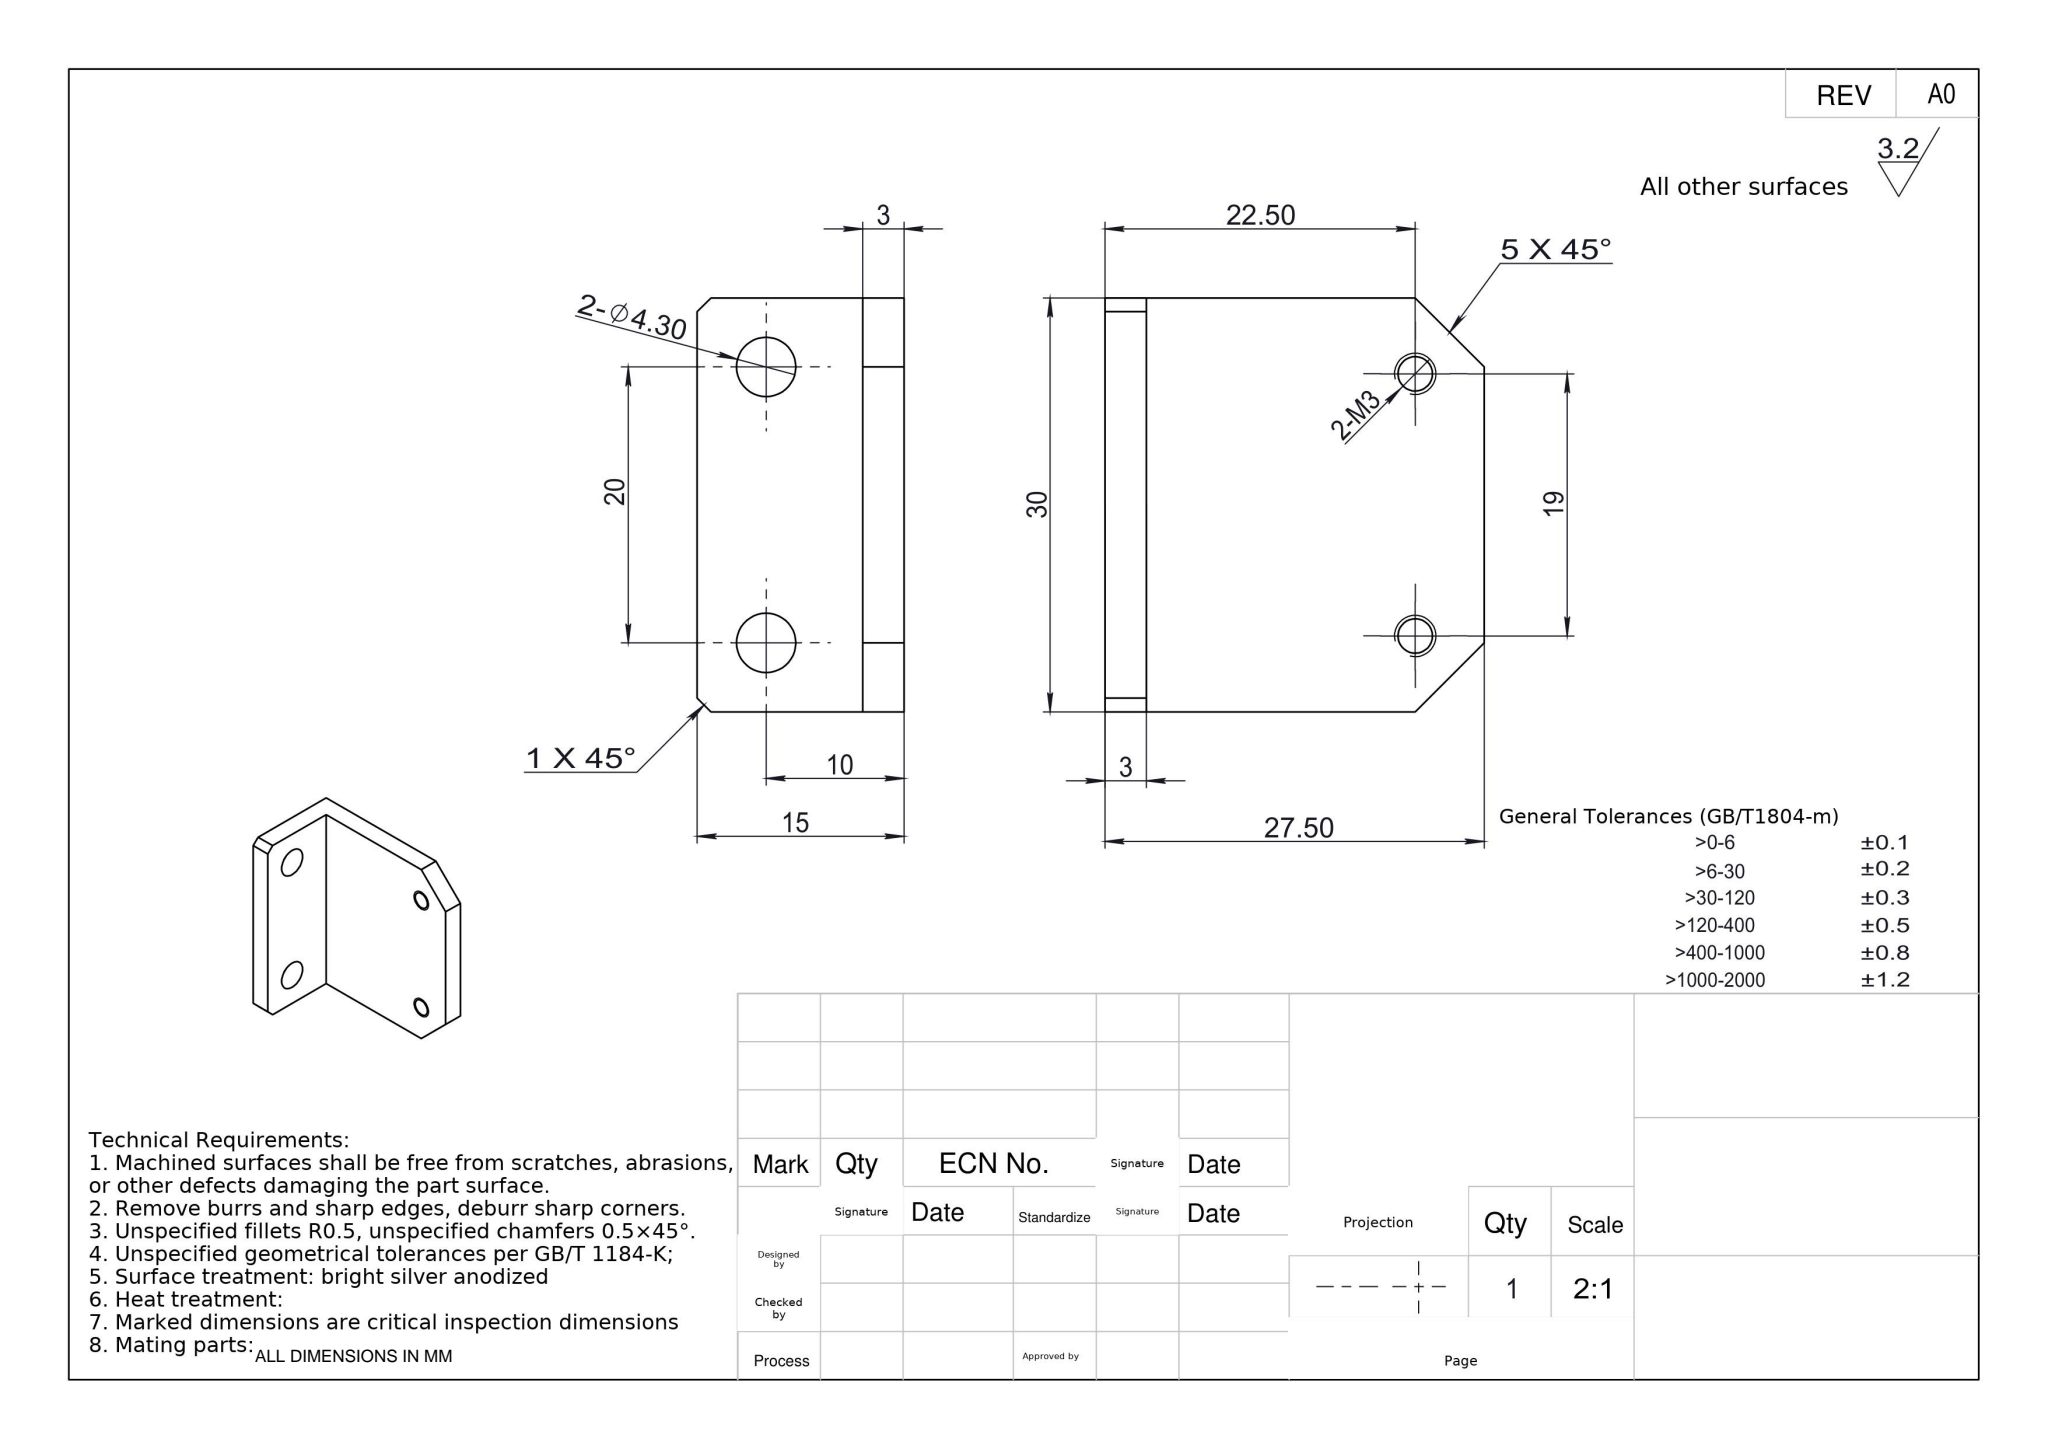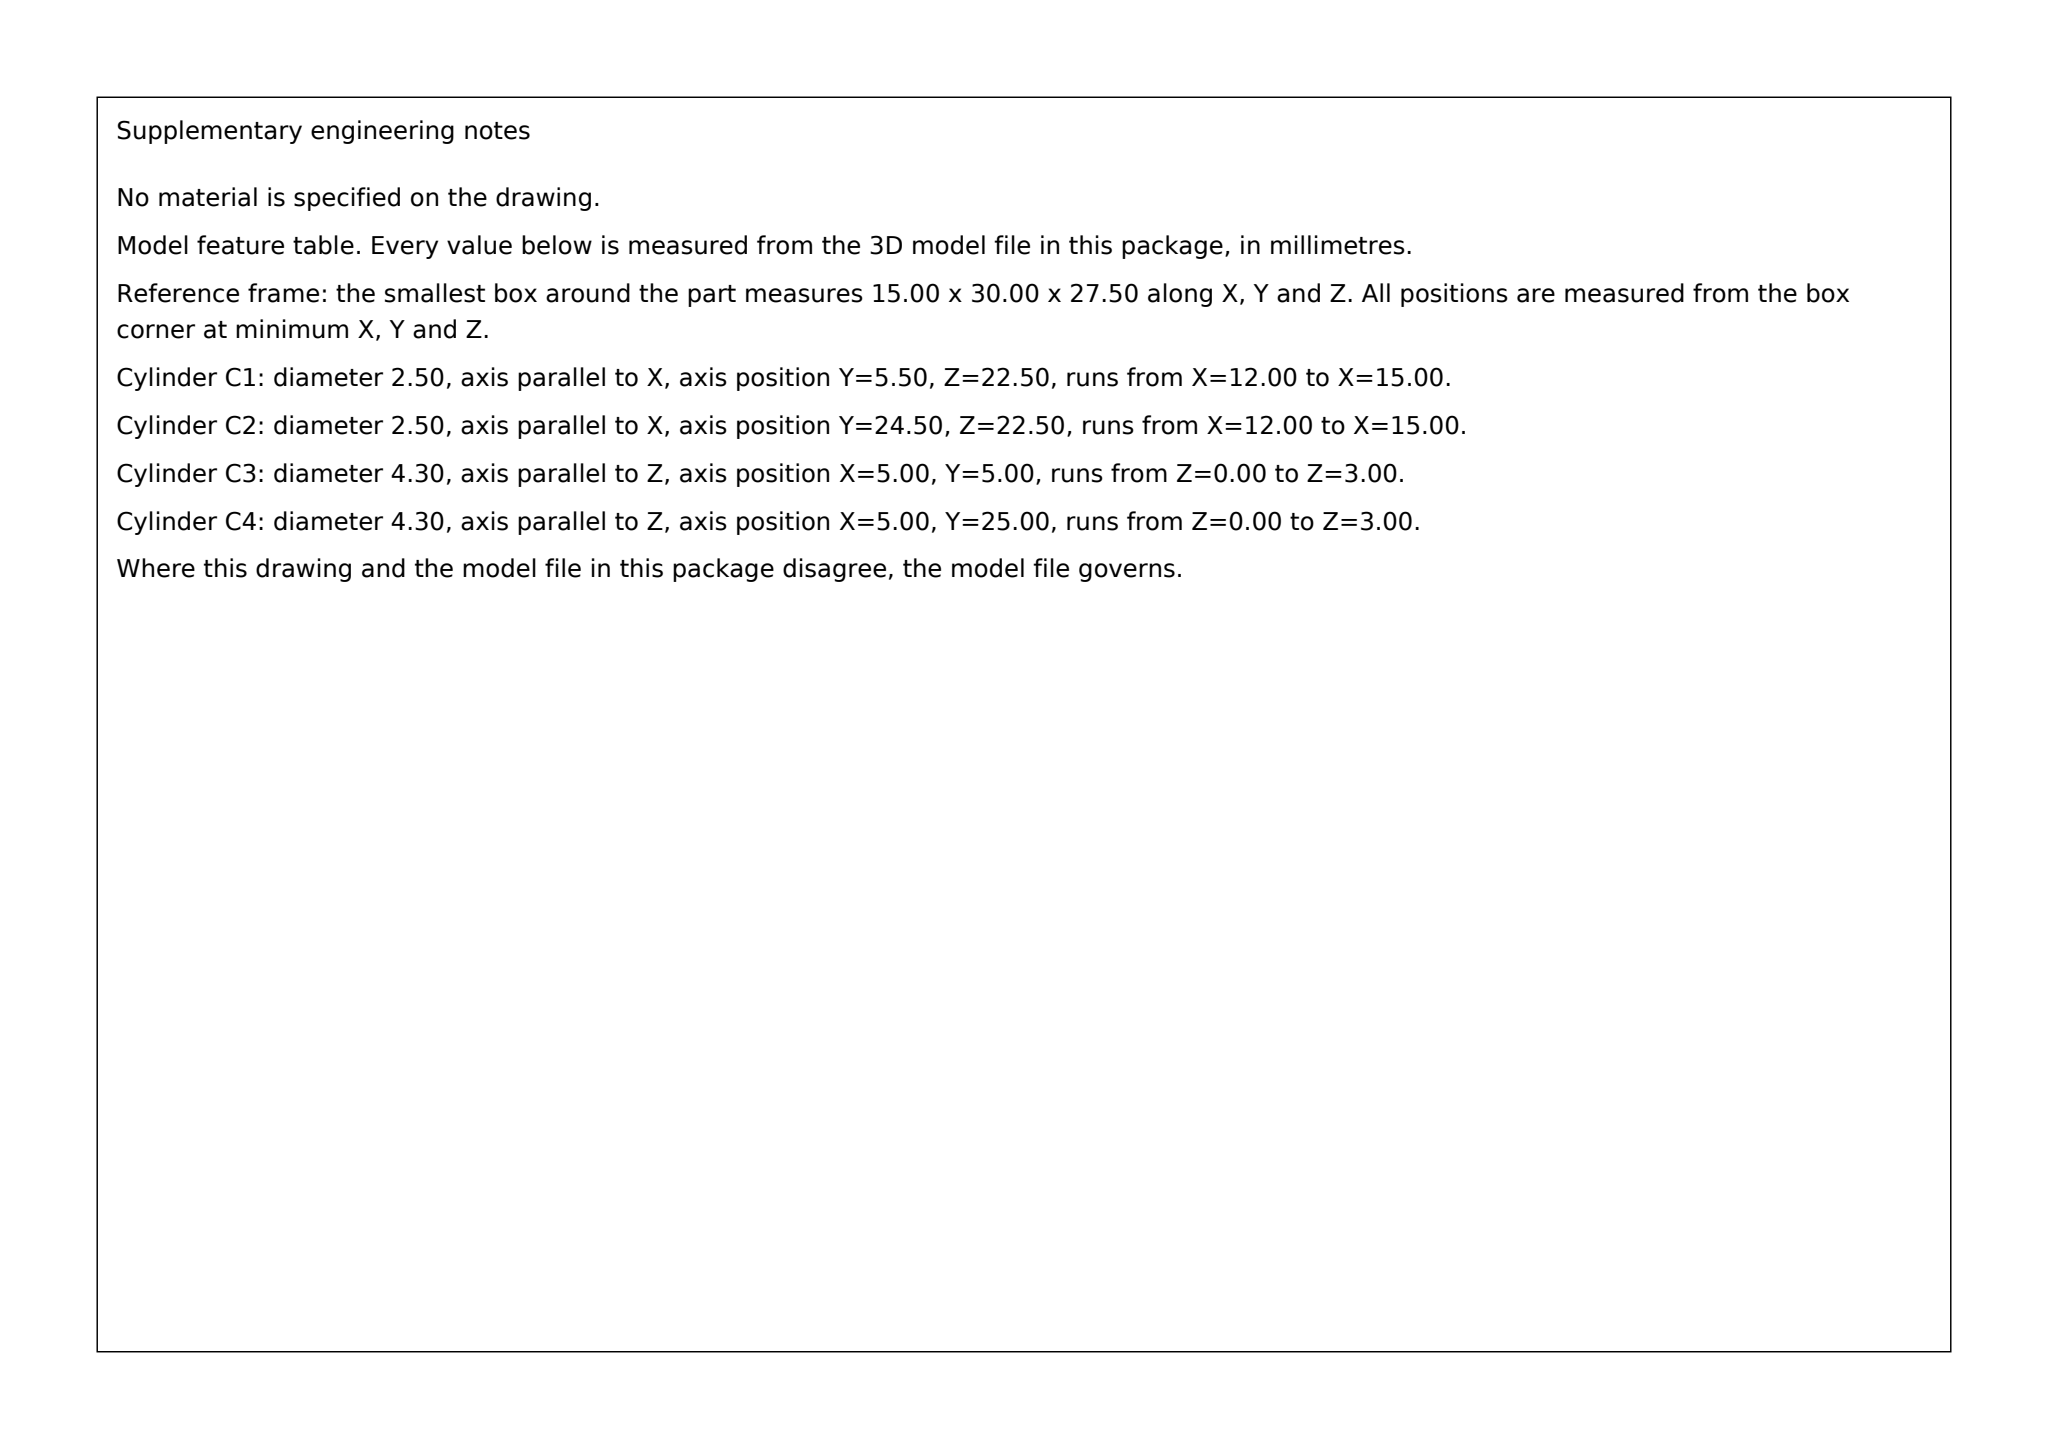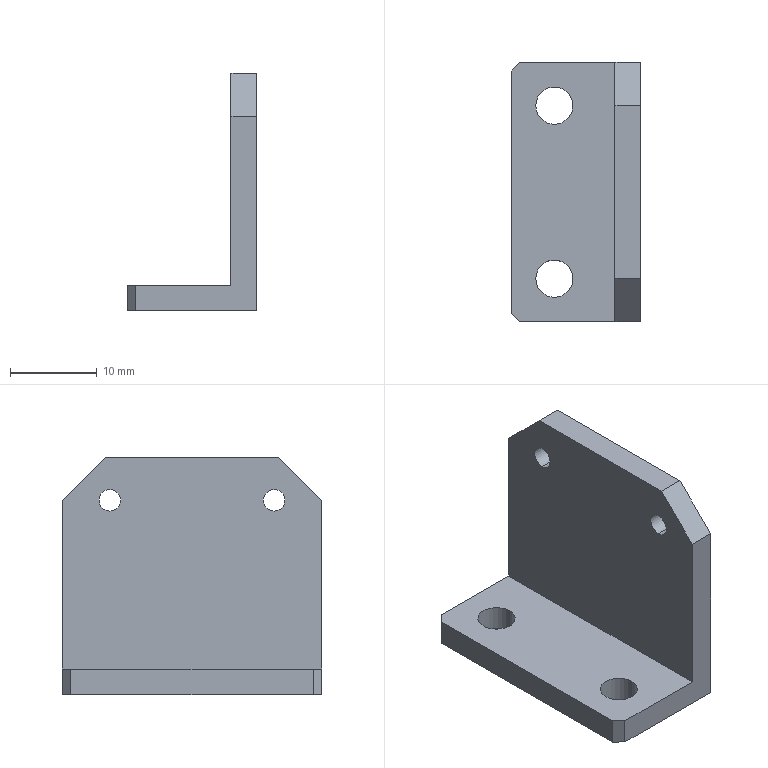Part | SolidWorks | mm | 1 solid | 20 faces | box 15 x 30 x 27.5 mm | volume 3360 mm3 | plane 12 | cylinder 8 | commonest cylinder face diameters 4.3 x4 2.5 x4
build123d program:
from build123d import *

# Parameters (mm, degrees)
SKETCH1_W                = 3
SKETCH1_H                = 30
EXTRUDE_THIN1_DEPTH      = 15
SKETCH3_W                = 3
SKETCH3_H                = 30
BOSS_EXTRUDE1_DEPTH      = 24.5
M3_TAPPED_HOLE1_D        = 2.5
M3_TAPPED_HOLE1_DEPTH    = 8.5
M3_TAPPED_HOLE1_TIP      = 0.7511
CHAMFER1_SIZE            = 5
M4_CLEARANCE_HOLE1_D     = 4.3
M4_CLEARANCE_HOLE1_DEPTH = 23
M4_CLEARANCE_HOLE1_TIP   = 1.292
CHAMFER2_SIZE            = 1


with BuildPart() as part:
    # Sketch1 → Extrude-Thin1 (new body)
    with BuildSketch(Plane(origin=(0, 0, 0), x_dir=(0, 0, -1), z_dir=(1, 0, 0))):
        with Locations((1.5, 15)):
            Rectangle(SKETCH1_W, SKETCH1_H)
    extrude(amount=EXTRUDE_THIN1_DEPTH)

    # Sketch3 → Boss-Extrude1 (add)
    with BuildSketch(Plane.XY):
        with Locations((13.5, 15)):
            Rectangle(SKETCH3_W, SKETCH3_H)
    extrude(amount=BOSS_EXTRUDE1_DEPTH)

    # M3 Tapped Hole1
    with Locations(Plane.ZY.offset(-12)):
        with Locations((19.5, 24.5), (19.5, 5.5)):
            Hole(M3_TAPPED_HOLE1_D / 2, depth=M3_TAPPED_HOLE1_DEPTH)
            with Locations((0, 0, -(M3_TAPPED_HOLE1_DEPTH + M3_TAPPED_HOLE1_TIP / 2))):  # 118° drill point
                Cone(0, M3_TAPPED_HOLE1_D / 2, M3_TAPPED_HOLE1_TIP, mode=Mode.SUBTRACT)

    # Chamfer1
    chamfer1_edges = [part.edges().sort_by_distance(p)[0] for p in [
        (13.5, 30, 24.5),
        (13.5, 0, 24.5),
    ]]
    chamfer(chamfer1_edges, length=CHAMFER1_SIZE)

    # M4 Clearance Hole1
    with Locations(Plane.XY):
        with Locations((5, 5), (5, 25)):
            Hole(M4_CLEARANCE_HOLE1_D / 2, depth=M4_CLEARANCE_HOLE1_DEPTH)
            with Locations((0, 0, -(M4_CLEARANCE_HOLE1_DEPTH + M4_CLEARANCE_HOLE1_TIP / 2))):  # 118° drill point
                Cone(0, M4_CLEARANCE_HOLE1_D / 2, M4_CLEARANCE_HOLE1_TIP, mode=Mode.SUBTRACT)

    # Chamfer2
    chamfer2_edges = [part.edges().sort_by_distance(p)[0] for p in [
        (0, 0, -1.5),
        (0, 30, -1.5),
    ]]
    chamfer(chamfer2_edges, length=CHAMFER2_SIZE)


solid = part.part
STEP:
#1=CARTESIAN_POINT('',(2.85,5.,-3.));
#2=VERTEX_POINT('',#1);
#3=CARTESIAN_POINT('',(7.15,5.,-3.));
#4=VERTEX_POINT('',#3);
#5=CARTESIAN_POINT('',(5.,5.,-3.));
#6=DIRECTION('',(0.,0.,1.));
#7=DIRECTION('',(1.,0.,0.));
#8=AXIS2_PLACEMENT_3D('',#5,#6,#7);
#9=CIRCLE('',#8,2.15);
#10=EDGE_CURVE('',#2,#4,#9,.T.);
#11=ORIENTED_EDGE('',*,*,#10,.F.);
#12=CARTESIAN_POINT('',(2.85,5.,-0.));
#13=VERTEX_POINT('',#12);
#14=CARTESIAN_POINT('',(2.85,5.,0.));
#15=DIRECTION('',(0.,0.,1.));
#16=VECTOR('',#15,1000.);
#17=LINE('',#14,#16);
#18=EDGE_CURVE('',#2,#13,#17,.T.);
#19=ORIENTED_EDGE('',*,*,#18,.T.);
#20=CARTESIAN_POINT('',(7.15,5.,-0.));
#21=VERTEX_POINT('',#20);
#22=CARTESIAN_POINT('',(5.,5.,-0.));
#23=DIRECTION('',(0.,0.,1.));
#24=DIRECTION('',(1.,0.,0.));
#25=AXIS2_PLACEMENT_3D('',#22,#23,#24);
#26=CIRCLE('',#25,2.15);
#27=EDGE_CURVE('',#13,#21,#26,.T.);
#28=ORIENTED_EDGE('',*,*,#27,.T.);
#29=CARTESIAN_POINT('',(7.15,5.,0.));
#30=DIRECTION('',(0.,0.,1.));
#31=VECTOR('',#30,1000.);
#32=LINE('',#29,#31);
#33=EDGE_CURVE('',#4,#21,#32,.T.);
#34=ORIENTED_EDGE('',*,*,#33,.F.);
#35=EDGE_LOOP('',(#11,#19,#28,#34));
#36=FACE_OUTER_BOUND('',#35,.T.);
#37=CARTESIAN_POINT('',(5.,5.,0.));
#38=DIRECTION('',(0.,0.,1.));
#39=DIRECTION('',(1.,0.,0.));
#40=AXIS2_PLACEMENT_3D('',#37,#38,#39);
#41=CYLINDRICAL_SURFACE('',#40,2.15);
#42=ADVANCED_FACE('',(#36),#41,.F.);
#43=CARTESIAN_POINT('',(2.85,25.,-3.));
#44=VERTEX_POINT('',#43);
#45=CARTESIAN_POINT('',(7.15,25.,-3.));
#46=VERTEX_POINT('',#45);
#47=CARTESIAN_POINT('',(5.,25.,-3.));
#48=DIRECTION('',(0.,0.,1.));
#49=DIRECTION('',(1.,0.,0.));
#50=AXIS2_PLACEMENT_3D('',#47,#48,#49);
#51=CIRCLE('',#50,2.15);
#52=EDGE_CURVE('',#44,#46,#51,.T.);
#53=ORIENTED_EDGE('',*,*,#52,.F.);
#54=CARTESIAN_POINT('',(2.85,25.,-0.));
#55=VERTEX_POINT('',#54);
#56=CARTESIAN_POINT('',(2.85,25.,0.));
#57=DIRECTION('',(0.,0.,1.));
#58=VECTOR('',#57,1000.);
#59=LINE('',#56,#58);
#60=EDGE_CURVE('',#44,#55,#59,.T.);
#61=ORIENTED_EDGE('',*,*,#60,.T.);
#62=CARTESIAN_POINT('',(7.15,25.,-0.));
#63=VERTEX_POINT('',#62);
#64=CARTESIAN_POINT('',(5.,25.,-0.));
#65=DIRECTION('',(0.,0.,1.));
#66=DIRECTION('',(1.,0.,0.));
#67=AXIS2_PLACEMENT_3D('',#64,#65,#66);
#68=CIRCLE('',#67,2.15);
#69=EDGE_CURVE('',#55,#63,#68,.T.);
#70=ORIENTED_EDGE('',*,*,#69,.T.);
#71=CARTESIAN_POINT('',(7.15,25.,0.));
#72=DIRECTION('',(0.,0.,1.));
#73=VECTOR('',#72,1000.);
#74=LINE('',#71,#73);
#75=EDGE_CURVE('',#46,#63,#74,.T.);
#76=ORIENTED_EDGE('',*,*,#75,.F.);
#77=EDGE_LOOP('',(#53,#61,#70,#76));
#78=FACE_OUTER_BOUND('',#77,.T.);
#79=CARTESIAN_POINT('',(5.,25.,0.));
#80=DIRECTION('',(0.,0.,1.));
#81=DIRECTION('',(1.,0.,0.));
#82=AXIS2_PLACEMENT_3D('',#79,#80,#81);
#83=CYLINDRICAL_SURFACE('',#82,2.15);
#84=ADVANCED_FACE('',(#78),#83,.F.);
#85=CARTESIAN_POINT('',(15.,24.5,18.25));
#86=VERTEX_POINT('',#85);
#87=CARTESIAN_POINT('',(15.,24.5,20.75));
#88=VERTEX_POINT('',#87);
#89=CARTESIAN_POINT('',(15.,24.5,19.5));
#90=DIRECTION('',(-1.,0.,0.));
#91=DIRECTION('',(0.,0.,1.));
#92=AXIS2_PLACEMENT_3D('',#89,#90,#91);
#93=CIRCLE('',#92,1.25);
#94=EDGE_CURVE('',#86,#88,#93,.T.);
#95=ORIENTED_EDGE('',*,*,#94,.F.);
#96=CARTESIAN_POINT('',(12.,24.5,18.25));
#97=VERTEX_POINT('',#96);
#98=CARTESIAN_POINT('',(12.,24.5,18.25));
#99=DIRECTION('',(-1.,0.,0.));
#100=VECTOR('',#99,1000.);
#101=LINE('',#98,#100);
#102=EDGE_CURVE('',#86,#97,#101,.T.);
#103=ORIENTED_EDGE('',*,*,#102,.T.);
#104=CARTESIAN_POINT('',(12.,24.5,20.75));
#105=VERTEX_POINT('',#104);
#106=CARTESIAN_POINT('',(12.,24.5,19.5));
#107=DIRECTION('',(-1.,0.,0.));
#108=DIRECTION('',(0.,0.,1.));
#109=AXIS2_PLACEMENT_3D('',#106,#107,#108);
#110=CIRCLE('',#109,1.25);
#111=EDGE_CURVE('',#97,#105,#110,.T.);
#112=ORIENTED_EDGE('',*,*,#111,.T.);
#113=CARTESIAN_POINT('',(12.,24.5,20.75));
#114=DIRECTION('',(-1.,0.,0.));
#115=VECTOR('',#114,1000.);
#116=LINE('',#113,#115);
#117=EDGE_CURVE('',#88,#105,#116,.T.);
#118=ORIENTED_EDGE('',*,*,#117,.F.);
#119=EDGE_LOOP('',(#95,#103,#112,#118));
#120=FACE_OUTER_BOUND('',#119,.T.);
#121=CARTESIAN_POINT('',(12.,24.5,19.5));
#122=DIRECTION('',(-1.,0.,0.));
#123=DIRECTION('',(0.,0.,1.));
#124=AXIS2_PLACEMENT_3D('',#121,#122,#123);
#125=CYLINDRICAL_SURFACE('',#124,1.25);
#126=ADVANCED_FACE('',(#120),#125,.F.);
#127=CARTESIAN_POINT('',(15.,5.5,18.25));
#128=VERTEX_POINT('',#127);
#129=CARTESIAN_POINT('',(15.,5.5,20.75));
#130=VERTEX_POINT('',#129);
#131=CARTESIAN_POINT('',(15.,5.5,19.5));
#132=DIRECTION('',(-1.,0.,0.));
#133=DIRECTION('',(0.,0.,1.));
#134=AXIS2_PLACEMENT_3D('',#131,#132,#133);
#135=CIRCLE('',#134,1.25);
#136=EDGE_CURVE('',#128,#130,#135,.T.);
#137=ORIENTED_EDGE('',*,*,#136,.F.);
#138=CARTESIAN_POINT('',(12.,5.5,18.25));
#139=VERTEX_POINT('',#138);
#140=CARTESIAN_POINT('',(12.,5.5,18.25));
#141=DIRECTION('',(-1.,0.,0.));
#142=VECTOR('',#141,1000.);
#143=LINE('',#140,#142);
#144=EDGE_CURVE('',#128,#139,#143,.T.);
#145=ORIENTED_EDGE('',*,*,#144,.T.);
#146=CARTESIAN_POINT('',(12.,5.5,20.75));
#147=VERTEX_POINT('',#146);
#148=CARTESIAN_POINT('',(12.,5.5,19.5));
#149=DIRECTION('',(-1.,0.,0.));
#150=DIRECTION('',(0.,0.,1.));
#151=AXIS2_PLACEMENT_3D('',#148,#149,#150);
#152=CIRCLE('',#151,1.25);
#153=EDGE_CURVE('',#139,#147,#152,.T.);
#154=ORIENTED_EDGE('',*,*,#153,.T.);
#155=CARTESIAN_POINT('',(12.,5.5,20.75));
#156=DIRECTION('',(-1.,0.,0.));
#157=VECTOR('',#156,1000.);
#158=LINE('',#155,#157);
#159=EDGE_CURVE('',#130,#147,#158,.T.);
#160=ORIENTED_EDGE('',*,*,#159,.F.);
#161=EDGE_LOOP('',(#137,#145,#154,#160));
#162=FACE_OUTER_BOUND('',#161,.T.);
#163=CARTESIAN_POINT('',(12.,5.5,19.5));
#164=DIRECTION('',(-1.,0.,0.));
#165=DIRECTION('',(0.,0.,1.));
#166=AXIS2_PLACEMENT_3D('',#163,#164,#165);
#167=CYLINDRICAL_SURFACE('',#166,1.25);
#168=ADVANCED_FACE('',(#162),#167,.F.);
#169=CARTESIAN_POINT('',(5.,5.,-3.));
#170=DIRECTION('',(0.,0.,1.));
#171=DIRECTION('',(1.,0.,0.));
#172=AXIS2_PLACEMENT_3D('',#169,#170,#171);
#173=CIRCLE('',#172,2.15);
#174=EDGE_CURVE('',#4,#2,#173,.T.);
#175=ORIENTED_EDGE('',*,*,#174,.T.);
#176=ORIENTED_EDGE('',*,*,#10,.T.);
#177=EDGE_LOOP('',(#175,#176));
#178=FACE_BOUND('',#177,.T.);
#179=CARTESIAN_POINT('',(5.,25.,-3.));
#180=DIRECTION('',(0.,0.,1.));
#181=DIRECTION('',(1.,0.,0.));
#182=AXIS2_PLACEMENT_3D('',#179,#180,#181);
#183=CIRCLE('',#182,2.15);
#184=EDGE_CURVE('',#46,#44,#183,.T.);
#185=ORIENTED_EDGE('',*,*,#184,.T.);
#186=ORIENTED_EDGE('',*,*,#52,.T.);
#187=EDGE_LOOP('',(#185,#186));
#188=FACE_BOUND('',#187,.T.);
#189=CARTESIAN_POINT('',(15.,0.,-3.));
#190=VERTEX_POINT('',#189);
#191=CARTESIAN_POINT('',(1.,-0.,-3.));
#192=VERTEX_POINT('',#191);
#193=CARTESIAN_POINT('',(15.,0.,-3.));
#194=DIRECTION('',(-1.,0.,0.));
#195=VECTOR('',#194,1000.);
#196=LINE('',#193,#195);
#197=EDGE_CURVE('',#190,#192,#196,.T.);
#198=ORIENTED_EDGE('',*,*,#197,.T.);
#199=CARTESIAN_POINT('',(0.,1.,-3.));
#200=VERTEX_POINT('',#199);
#201=CARTESIAN_POINT('',(0.,1.,-3.));
#202=DIRECTION('',(-0.7071,0.7071,0.));
#203=VECTOR('',#202,1000.);
#204=LINE('',#201,#203);
#205=EDGE_CURVE('',#192,#200,#204,.T.);
#206=ORIENTED_EDGE('',*,*,#205,.T.);
#207=CARTESIAN_POINT('',(-0.,29.,-3.));
#208=VERTEX_POINT('',#207);
#209=CARTESIAN_POINT('',(0.,0.,-3.));
#210=DIRECTION('',(0.,1.,0.));
#211=VECTOR('',#210,1000.);
#212=LINE('',#209,#211);
#213=EDGE_CURVE('',#200,#208,#212,.T.);
#214=ORIENTED_EDGE('',*,*,#213,.T.);
#215=CARTESIAN_POINT('',(1.,30.,-3.));
#216=VERTEX_POINT('',#215);
#217=CARTESIAN_POINT('',(0.,29.,-3.));
#218=DIRECTION('',(0.7071,0.7071,0.));
#219=VECTOR('',#218,1000.);
#220=LINE('',#217,#219);
#221=EDGE_CURVE('',#208,#216,#220,.T.);
#222=ORIENTED_EDGE('',*,*,#221,.T.);
#223=CARTESIAN_POINT('',(15.,30.,-3.));
#224=VERTEX_POINT('',#223);
#225=CARTESIAN_POINT('',(15.,30.,-3.));
#226=DIRECTION('',(-1.,0.,0.));
#227=VECTOR('',#226,1000.);
#228=LINE('',#225,#227);
#229=EDGE_CURVE('',#224,#216,#228,.T.);
#230=ORIENTED_EDGE('',*,*,#229,.F.);
#231=CARTESIAN_POINT('',(15.,0.,-3.));
#232=DIRECTION('',(0.,1.,0.));
#233=VECTOR('',#232,1000.);
#234=LINE('',#231,#233);
#235=EDGE_CURVE('',#190,#224,#234,.T.);
#236=ORIENTED_EDGE('',*,*,#235,.F.);
#237=EDGE_LOOP('',(#198,#206,#214,#222,#230,#236));
#238=FACE_OUTER_BOUND('',#237,.T.);
#239=CARTESIAN_POINT('',(15.,0.,-3.));
#240=DIRECTION('',(0.,0.,1.));
#241=DIRECTION('',(1.,0.,0.));
#242=AXIS2_PLACEMENT_3D('',#239,#240,#241);
#243=PLANE('',#242);
#244=ADVANCED_FACE('',(#178,#188,#238),#243,.F.);
#245=ORIENTED_EDGE('',*,*,#229,.T.);
#246=CARTESIAN_POINT('',(1.,30.,0.));
#247=VERTEX_POINT('',#246);
#248=CARTESIAN_POINT('',(1.,30.,0.));
#249=DIRECTION('',(0.,0.,1.));
#250=VECTOR('',#249,1000.);
#251=LINE('',#248,#250);
#252=EDGE_CURVE('',#216,#247,#251,.T.);
#253=ORIENTED_EDGE('',*,*,#252,.T.);
#254=CARTESIAN_POINT('',(12.,30.,0.));
#255=VERTEX_POINT('',#254);
#256=CARTESIAN_POINT('',(15.,30.,0.));
#257=DIRECTION('',(-1.,0.,0.));
#258=VECTOR('',#257,1000.);
#259=LINE('',#256,#258);
#260=EDGE_CURVE('',#255,#247,#259,.T.);
#261=ORIENTED_EDGE('',*,*,#260,.F.);
#262=CARTESIAN_POINT('',(12.,30.,19.5));
#263=VERTEX_POINT('',#262);
#264=CARTESIAN_POINT('',(12.,30.,24.5));
#265=DIRECTION('',(0.,0.,-1.));
#266=VECTOR('',#265,1000.);
#267=LINE('',#264,#266);
#268=EDGE_CURVE('',#263,#255,#267,.T.);
#269=ORIENTED_EDGE('',*,*,#268,.F.);
#270=CARTESIAN_POINT('',(15.,30.,19.5));
#271=VERTEX_POINT('',#270);
#272=CARTESIAN_POINT('',(15.,30.,19.5));
#273=DIRECTION('',(1.,0.,0.));
#274=VECTOR('',#273,1000.);
#275=LINE('',#272,#274);
#276=EDGE_CURVE('',#263,#271,#275,.T.);
#277=ORIENTED_EDGE('',*,*,#276,.T.);
#278=CARTESIAN_POINT('',(15.,30.,0.));
#279=DIRECTION('',(0.,0.,-1.));
#280=VECTOR('',#279,1000.);
#281=LINE('',#278,#280);
#282=EDGE_CURVE('',#271,#224,#281,.T.);
#283=ORIENTED_EDGE('',*,*,#282,.T.);
#284=EDGE_LOOP('',(#245,#253,#261,#269,#277,#283));
#285=FACE_OUTER_BOUND('',#284,.T.);
#286=CARTESIAN_POINT('',(15.,30.,0.));
#287=DIRECTION('',(0.,1.,0.));
#288=DIRECTION('',(0.,0.,1.));
#289=AXIS2_PLACEMENT_3D('',#286,#287,#288);
#290=PLANE('',#289);
#291=ADVANCED_FACE('',(#285),#290,.T.);
#292=CARTESIAN_POINT('',(5.,5.,-0.));
#293=DIRECTION('',(0.,0.,1.));
#294=DIRECTION('',(1.,0.,0.));
#295=AXIS2_PLACEMENT_3D('',#292,#293,#294);
#296=CIRCLE('',#295,2.15);
#297=EDGE_CURVE('',#21,#13,#296,.T.);
#298=ORIENTED_EDGE('',*,*,#297,.F.);
#299=ORIENTED_EDGE('',*,*,#27,.F.);
#300=EDGE_LOOP('',(#298,#299));
#301=FACE_BOUND('',#300,.T.);
#302=CARTESIAN_POINT('',(5.,25.,-0.));
#303=DIRECTION('',(0.,0.,1.));
#304=DIRECTION('',(1.,0.,0.));
#305=AXIS2_PLACEMENT_3D('',#302,#303,#304);
#306=CIRCLE('',#305,2.15);
#307=EDGE_CURVE('',#63,#55,#306,.T.);
#308=ORIENTED_EDGE('',*,*,#307,.F.);
#309=ORIENTED_EDGE('',*,*,#69,.F.);
#310=EDGE_LOOP('',(#308,#309));
#311=FACE_BOUND('',#310,.T.);
#312=CARTESIAN_POINT('',(-0.,1.,0.));
#313=VERTEX_POINT('',#312);
#314=CARTESIAN_POINT('',(-0.,29.,0.));
#315=VERTEX_POINT('',#314);
#316=CARTESIAN_POINT('',(0.,0.,0.));
#317=DIRECTION('',(0.,1.,0.));
#318=VECTOR('',#317,1000.);
#319=LINE('',#316,#318);
#320=EDGE_CURVE('',#313,#315,#319,.T.);
#321=ORIENTED_EDGE('',*,*,#320,.F.);
#322=CARTESIAN_POINT('',(1.,0.,0.));
#323=VERTEX_POINT('',#322);
#324=CARTESIAN_POINT('',(8.,-7.,0.));
#325=DIRECTION('',(0.7071,-0.7071,0.));
#326=VECTOR('',#325,1000.);
#327=LINE('',#324,#326);
#328=EDGE_CURVE('',#313,#323,#327,.T.);
#329=ORIENTED_EDGE('',*,*,#328,.T.);
#330=CARTESIAN_POINT('',(12.,0.,0.));
#331=VERTEX_POINT('',#330);
#332=CARTESIAN_POINT('',(15.,0.,0.));
#333=DIRECTION('',(-1.,0.,0.));
#334=VECTOR('',#333,1000.);
#335=LINE('',#332,#334);
#336=EDGE_CURVE('',#331,#323,#335,.T.);
#337=ORIENTED_EDGE('',*,*,#336,.F.);
#338=CARTESIAN_POINT('',(12.,30.,0.));
#339=DIRECTION('',(0.,-1.,0.));
#340=VECTOR('',#339,1000.);
#341=LINE('',#338,#340);
#342=EDGE_CURVE('',#255,#331,#341,.T.);
#343=ORIENTED_EDGE('',*,*,#342,.F.);
#344=ORIENTED_EDGE('',*,*,#260,.T.);
#345=CARTESIAN_POINT('',(-7.,22.,0.));
#346=DIRECTION('',(-0.7071,-0.7071,0.));
#347=VECTOR('',#346,1000.);
#348=LINE('',#345,#347);
#349=EDGE_CURVE('',#247,#315,#348,.T.);
#350=ORIENTED_EDGE('',*,*,#349,.T.);
#351=EDGE_LOOP('',(#321,#329,#337,#343,#344,#350));
#352=FACE_OUTER_BOUND('',#351,.T.);
#353=CARTESIAN_POINT('',(15.,0.,0.));
#354=DIRECTION('',(0.,0.,1.));
#355=DIRECTION('',(1.,0.,0.));
#356=AXIS2_PLACEMENT_3D('',#353,#354,#355);
#357=PLANE('',#356);
#358=ADVANCED_FACE('',(#301,#311,#352),#357,.T.);
#359=ORIENTED_EDGE('',*,*,#336,.T.);
#360=CARTESIAN_POINT('',(1.,0.,-3.));
#361=DIRECTION('',(0.,0.,-1.));
#362=VECTOR('',#361,1000.);
#363=LINE('',#360,#362);
#364=EDGE_CURVE('',#323,#192,#363,.T.);
#365=ORIENTED_EDGE('',*,*,#364,.T.);
#366=ORIENTED_EDGE('',*,*,#197,.F.);
#367=CARTESIAN_POINT('',(15.,0.,19.5));
#368=VERTEX_POINT('',#367);
#369=CARTESIAN_POINT('',(15.,0.,-3.));
#370=DIRECTION('',(0.,0.,1.));
#371=VECTOR('',#370,1000.);
#372=LINE('',#369,#371);
#373=EDGE_CURVE('',#190,#368,#372,.T.);
#374=ORIENTED_EDGE('',*,*,#373,.T.);
#375=CARTESIAN_POINT('',(12.,0.,19.5));
#376=VERTEX_POINT('',#375);
#377=CARTESIAN_POINT('',(15.,0.,19.5));
#378=DIRECTION('',(-1.,0.,0.));
#379=VECTOR('',#378,1000.);
#380=LINE('',#377,#379);
#381=EDGE_CURVE('',#368,#376,#380,.T.);
#382=ORIENTED_EDGE('',*,*,#381,.T.);
#383=CARTESIAN_POINT('',(12.,0.,24.5));
#384=DIRECTION('',(0.,0.,-1.));
#385=VECTOR('',#384,1000.);
#386=LINE('',#383,#385);
#387=EDGE_CURVE('',#376,#331,#386,.T.);
#388=ORIENTED_EDGE('',*,*,#387,.T.);
#389=EDGE_LOOP('',(#359,#365,#366,#374,#382,#388));
#390=FACE_OUTER_BOUND('',#389,.T.);
#391=CARTESIAN_POINT('',(15.,0.,-3.));
#392=DIRECTION('',(0.,-1.,0.));
#393=DIRECTION('',(0.,0.,-1.));
#394=AXIS2_PLACEMENT_3D('',#391,#392,#393);
#395=PLANE('',#394);
#396=ADVANCED_FACE('',(#390),#395,.T.);
#397=CARTESIAN_POINT('',(15.,24.5,19.5));
#398=DIRECTION('',(-1.,0.,0.));
#399=DIRECTION('',(0.,0.,1.));
#400=AXIS2_PLACEMENT_3D('',#397,#398,#399);
#401=CIRCLE('',#400,1.25);
#402=EDGE_CURVE('',#88,#86,#401,.T.);
#403=ORIENTED_EDGE('',*,*,#402,.T.);
#404=ORIENTED_EDGE('',*,*,#94,.T.);
#405=EDGE_LOOP('',(#403,#404));
#406=FACE_BOUND('',#405,.T.);
#407=CARTESIAN_POINT('',(15.,5.5,19.5));
#408=DIRECTION('',(-1.,0.,0.));
#409=DIRECTION('',(0.,0.,1.));
#410=AXIS2_PLACEMENT_3D('',#407,#408,#409);
#411=CIRCLE('',#410,1.25);
#412=EDGE_CURVE('',#130,#128,#411,.T.);
#413=ORIENTED_EDGE('',*,*,#412,.T.);
#414=ORIENTED_EDGE('',*,*,#136,.T.);
#415=EDGE_LOOP('',(#413,#414));
#416=FACE_BOUND('',#415,.T.);
#417=ORIENTED_EDGE('',*,*,#282,.F.);
#418=CARTESIAN_POINT('',(15.,25.,24.5));
#419=VERTEX_POINT('',#418);
#420=CARTESIAN_POINT('',(15.,25.,24.5));
#421=DIRECTION('',(0.,-0.7071,0.7071));
#422=VECTOR('',#421,1000.);
#423=LINE('',#420,#422);
#424=EDGE_CURVE('',#271,#419,#423,.T.);
#425=ORIENTED_EDGE('',*,*,#424,.T.);
#426=CARTESIAN_POINT('',(15.,5.,24.5));
#427=VERTEX_POINT('',#426);
#428=CARTESIAN_POINT('',(15.,30.,24.5));
#429=DIRECTION('',(-0.,1.,0.));
#430=VECTOR('',#429,1000.);
#431=LINE('',#428,#430);
#432=EDGE_CURVE('',#427,#419,#431,.T.);
#433=ORIENTED_EDGE('',*,*,#432,.F.);
#434=CARTESIAN_POINT('',(15.,5.,24.5));
#435=DIRECTION('',(0.,-0.7071,-0.7071));
#436=VECTOR('',#435,1000.);
#437=LINE('',#434,#436);
#438=EDGE_CURVE('',#427,#368,#437,.T.);
#439=ORIENTED_EDGE('',*,*,#438,.T.);
#440=ORIENTED_EDGE('',*,*,#373,.F.);
#441=ORIENTED_EDGE('',*,*,#235,.T.);
#442=EDGE_LOOP('',(#417,#425,#433,#439,#440,#441));
#443=FACE_OUTER_BOUND('',#442,.T.);
#444=CARTESIAN_POINT('',(15.,0.,0.));
#445=DIRECTION('',(-1.,0.,0.));
#446=DIRECTION('',(0.,0.,1.));
#447=AXIS2_PLACEMENT_3D('',#444,#445,#446);
#448=PLANE('',#447);
#449=ADVANCED_FACE('',(#406,#416,#443),#448,.F.);
#450=ORIENTED_EDGE('',*,*,#213,.F.);
#451=CARTESIAN_POINT('',(0.,1.,0.));
#452=DIRECTION('',(0.,0.,1.));
#453=VECTOR('',#452,1000.);
#454=LINE('',#451,#453);
#455=EDGE_CURVE('',#200,#313,#454,.T.);
#456=ORIENTED_EDGE('',*,*,#455,.T.);
#457=ORIENTED_EDGE('',*,*,#320,.T.);
#458=CARTESIAN_POINT('',(0.,29.,0.));
#459=DIRECTION('',(0.,0.,-1.));
#460=VECTOR('',#459,1000.);
#461=LINE('',#458,#460);
#462=EDGE_CURVE('',#315,#208,#461,.T.);
#463=ORIENTED_EDGE('',*,*,#462,.T.);
#464=EDGE_LOOP('',(#450,#456,#457,#463));
#465=FACE_OUTER_BOUND('',#464,.T.);
#466=CARTESIAN_POINT('',(0.,0.,0.));
#467=DIRECTION('',(-1.,0.,0.));
#468=DIRECTION('',(0.,0.,1.));
#469=AXIS2_PLACEMENT_3D('',#466,#467,#468);
#470=PLANE('',#469);
#471=ADVANCED_FACE('',(#465),#470,.T.);
#472=CARTESIAN_POINT('',(12.,24.5,19.5));
#473=DIRECTION('',(-1.,0.,0.));
#474=DIRECTION('',(0.,0.,1.));
#475=AXIS2_PLACEMENT_3D('',#472,#473,#474);
#476=CIRCLE('',#475,1.25);
#477=EDGE_CURVE('',#105,#97,#476,.T.);
#478=ORIENTED_EDGE('',*,*,#477,.F.);
#479=ORIENTED_EDGE('',*,*,#111,.F.);
#480=EDGE_LOOP('',(#478,#479));
#481=FACE_BOUND('',#480,.T.);
#482=CARTESIAN_POINT('',(12.,5.5,19.5));
#483=DIRECTION('',(-1.,0.,0.));
#484=DIRECTION('',(0.,0.,1.));
#485=AXIS2_PLACEMENT_3D('',#482,#483,#484);
#486=CIRCLE('',#485,1.25);
#487=EDGE_CURVE('',#147,#139,#486,.T.);
#488=ORIENTED_EDGE('',*,*,#487,.F.);
#489=ORIENTED_EDGE('',*,*,#153,.F.);
#490=EDGE_LOOP('',(#488,#489));
#491=FACE_BOUND('',#490,.T.);
#492=CARTESIAN_POINT('',(12.,25.,24.5));
#493=VERTEX_POINT('',#492);
#494=CARTESIAN_POINT('',(12.,5.,24.5));
#495=VERTEX_POINT('',#494);
#496=CARTESIAN_POINT('',(12.,30.,24.5));
#497=DIRECTION('',(0.,-1.,0.));
#498=VECTOR('',#497,1000.);
#499=LINE('',#496,#498);
#500=EDGE_CURVE('',#493,#495,#499,.T.);
#501=ORIENTED_EDGE('',*,*,#500,.F.);
#502=CARTESIAN_POINT('',(12.,25.,24.5));
#503=DIRECTION('',(-0.,0.7071,-0.7071));
#504=VECTOR('',#503,1000.);
#505=LINE('',#502,#504);
#506=EDGE_CURVE('',#493,#263,#505,.T.);
#507=ORIENTED_EDGE('',*,*,#506,.T.);
#508=ORIENTED_EDGE('',*,*,#268,.T.);
#509=ORIENTED_EDGE('',*,*,#342,.T.);
#510=ORIENTED_EDGE('',*,*,#387,.F.);
#511=CARTESIAN_POINT('',(12.,5.,24.5));
#512=DIRECTION('',(-0.,0.7071,0.7071));
#513=VECTOR('',#512,1000.);
#514=LINE('',#511,#513);
#515=EDGE_CURVE('',#376,#495,#514,.T.);
#516=ORIENTED_EDGE('',*,*,#515,.T.);
#517=EDGE_LOOP('',(#501,#507,#508,#509,#510,#516));
#518=FACE_OUTER_BOUND('',#517,.T.);
#519=CARTESIAN_POINT('',(12.,30.,24.5));
#520=DIRECTION('',(1.,0.,0.));
#521=DIRECTION('',(-0.,1.,0.));
#522=AXIS2_PLACEMENT_3D('',#519,#520,#521);
#523=PLANE('',#522);
#524=ADVANCED_FACE('',(#481,#491,#518),#523,.F.);
#525=ORIENTED_EDGE('',*,*,#432,.T.);
#526=CARTESIAN_POINT('',(0.,25.,24.5));
#527=DIRECTION('',(-1.,0.,0.));
#528=VECTOR('',#527,1000.);
#529=LINE('',#526,#528);
#530=EDGE_CURVE('',#419,#493,#529,.T.);
#531=ORIENTED_EDGE('',*,*,#530,.T.);
#532=ORIENTED_EDGE('',*,*,#500,.T.);
#533=CARTESIAN_POINT('',(0.,5.,24.5));
#534=DIRECTION('',(1.,0.,0.));
#535=VECTOR('',#534,1000.);
#536=LINE('',#533,#535);
#537=EDGE_CURVE('',#495,#427,#536,.T.);
#538=ORIENTED_EDGE('',*,*,#537,.T.);
#539=EDGE_LOOP('',(#525,#531,#532,#538));
#540=FACE_OUTER_BOUND('',#539,.T.);
#541=CARTESIAN_POINT('',(0.,0.,24.5));
#542=DIRECTION('',(0.,0.,1.));
#543=DIRECTION('',(1.,0.,0.));
#544=AXIS2_PLACEMENT_3D('',#541,#542,#543);
#545=PLANE('',#544);
#546=ADVANCED_FACE('',(#540),#545,.T.);
#547=ORIENTED_EDGE('',*,*,#144,.F.);
#548=ORIENTED_EDGE('',*,*,#412,.F.);
#549=ORIENTED_EDGE('',*,*,#159,.T.);
#550=ORIENTED_EDGE('',*,*,#487,.T.);
#551=EDGE_LOOP('',(#547,#548,#549,#550));
#552=FACE_OUTER_BOUND('',#551,.T.);
#553=CARTESIAN_POINT('',(12.,5.5,19.5));
#554=DIRECTION('',(-1.,0.,0.));
#555=DIRECTION('',(0.,0.,1.));
#556=AXIS2_PLACEMENT_3D('',#553,#554,#555);
#557=CYLINDRICAL_SURFACE('',#556,1.25);
#558=ADVANCED_FACE('',(#552),#557,.F.);
#559=ORIENTED_EDGE('',*,*,#102,.F.);
#560=ORIENTED_EDGE('',*,*,#402,.F.);
#561=ORIENTED_EDGE('',*,*,#117,.T.);
#562=ORIENTED_EDGE('',*,*,#477,.T.);
#563=EDGE_LOOP('',(#559,#560,#561,#562));
#564=FACE_OUTER_BOUND('',#563,.T.);
#565=CARTESIAN_POINT('',(12.,24.5,19.5));
#566=DIRECTION('',(-1.,0.,0.));
#567=DIRECTION('',(0.,0.,1.));
#568=AXIS2_PLACEMENT_3D('',#565,#566,#567);
#569=CYLINDRICAL_SURFACE('',#568,1.25);
#570=ADVANCED_FACE('',(#564),#569,.F.);
#571=ORIENTED_EDGE('',*,*,#424,.F.);
#572=ORIENTED_EDGE('',*,*,#276,.F.);
#573=ORIENTED_EDGE('',*,*,#506,.F.);
#574=ORIENTED_EDGE('',*,*,#530,.F.);
#575=EDGE_LOOP('',(#571,#572,#573,#574));
#576=FACE_OUTER_BOUND('',#575,.T.);
#577=CARTESIAN_POINT('',(0.,25.,24.5));
#578=DIRECTION('',(0.,-0.7071,-0.7071));
#579=DIRECTION('',(-1.,0.,0.));
#580=AXIS2_PLACEMENT_3D('',#577,#578,#579);
#581=PLANE('',#580);
#582=ADVANCED_FACE('',(#576),#581,.F.);
#583=ORIENTED_EDGE('',*,*,#515,.F.);
#584=ORIENTED_EDGE('',*,*,#381,.F.);
#585=ORIENTED_EDGE('',*,*,#438,.F.);
#586=ORIENTED_EDGE('',*,*,#537,.F.);
#587=EDGE_LOOP('',(#583,#584,#585,#586));
#588=FACE_OUTER_BOUND('',#587,.T.);
#589=CARTESIAN_POINT('',(0.,5.,24.5));
#590=DIRECTION('',(0.,0.7071,-0.7071));
#591=DIRECTION('',(1.,0.,0.));
#592=AXIS2_PLACEMENT_3D('',#589,#590,#591);
#593=PLANE('',#592);
#594=ADVANCED_FACE('',(#588),#593,.F.);
#595=ORIENTED_EDGE('',*,*,#60,.F.);
#596=ORIENTED_EDGE('',*,*,#184,.F.);
#597=ORIENTED_EDGE('',*,*,#75,.T.);
#598=ORIENTED_EDGE('',*,*,#307,.T.);
#599=EDGE_LOOP('',(#595,#596,#597,#598));
#600=FACE_OUTER_BOUND('',#599,.T.);
#601=CARTESIAN_POINT('',(5.,25.,0.));
#602=DIRECTION('',(0.,0.,1.));
#603=DIRECTION('',(1.,0.,0.));
#604=AXIS2_PLACEMENT_3D('',#601,#602,#603);
#605=CYLINDRICAL_SURFACE('',#604,2.15);
#606=ADVANCED_FACE('',(#600),#605,.F.);
#607=ORIENTED_EDGE('',*,*,#18,.F.);
#608=ORIENTED_EDGE('',*,*,#174,.F.);
#609=ORIENTED_EDGE('',*,*,#33,.T.);
#610=ORIENTED_EDGE('',*,*,#297,.T.);
#611=EDGE_LOOP('',(#607,#608,#609,#610));
#612=FACE_OUTER_BOUND('',#611,.T.);
#613=CARTESIAN_POINT('',(5.,5.,0.));
#614=DIRECTION('',(0.,0.,1.));
#615=DIRECTION('',(1.,0.,0.));
#616=AXIS2_PLACEMENT_3D('',#613,#614,#615);
#617=CYLINDRICAL_SURFACE('',#616,2.15);
#618=ADVANCED_FACE('',(#612),#617,.F.);
#619=ORIENTED_EDGE('',*,*,#205,.F.);
#620=ORIENTED_EDGE('',*,*,#364,.F.);
#621=ORIENTED_EDGE('',*,*,#328,.F.);
#622=ORIENTED_EDGE('',*,*,#455,.F.);
#623=EDGE_LOOP('',(#619,#620,#621,#622));
#624=FACE_OUTER_BOUND('',#623,.T.);
#625=CARTESIAN_POINT('',(0.,1.,0.));
#626=DIRECTION('',(0.7071,0.7071,0.));
#627=DIRECTION('',(0.,0.,1.));
#628=AXIS2_PLACEMENT_3D('',#625,#626,#627);
#629=PLANE('',#628);
#630=ADVANCED_FACE('',(#624),#629,.F.);
#631=ORIENTED_EDGE('',*,*,#349,.F.);
#632=ORIENTED_EDGE('',*,*,#252,.F.);
#633=ORIENTED_EDGE('',*,*,#221,.F.);
#634=ORIENTED_EDGE('',*,*,#462,.F.);
#635=EDGE_LOOP('',(#631,#632,#633,#634));
#636=FACE_OUTER_BOUND('',#635,.T.);
#637=CARTESIAN_POINT('',(0.,29.,0.));
#638=DIRECTION('',(0.7071,-0.7071,0.));
#639=DIRECTION('',(0.,0.,-1.));
#640=AXIS2_PLACEMENT_3D('',#637,#638,#639);
#641=PLANE('',#640);
#642=ADVANCED_FACE('',(#636),#641,.F.);
#643=CLOSED_SHELL('',(#42,#84,#126,#168,#244,#291,#358,#396,#449,#471,#524,#546,#558,#570,#582,#594,#606,#618,#630,#642));
#644=MANIFOLD_SOLID_BREP('',#643);
#645=CARTESIAN_POINT('',(0.,0.,0.));
#646=DIRECTION('',(0.,0.,1.));
#647=DIRECTION('',(1.,0.,0.));
#648=AXIS2_PLACEMENT_3D('',#645,#646,#647);
#649=(LENGTH_UNIT()NAMED_UNIT(*)SI_UNIT(.MILLI.,.METRE.));
#650=UNCERTAINTY_MEASURE_WITH_UNIT(LENGTH_MEASURE(0.00001),#649,'','');
#651=(NAMED_UNIT(*)PLANE_ANGLE_UNIT()SI_UNIT($,.RADIAN.));
#652=(NAMED_UNIT(*)SI_UNIT($,.STERADIAN.)SOLID_ANGLE_UNIT());
#653=(GEOMETRIC_REPRESENTATION_CONTEXT(3)GLOBAL_UNCERTAINTY_ASSIGNED_CONTEXT((#650))GLOBAL_UNIT_ASSIGNED_CONTEXT((#649,#651,#652))REPRESENTATION_CONTEXT('',''));
#654=ADVANCED_BREP_SHAPE_REPRESENTATION('',(#644,#648),#653);